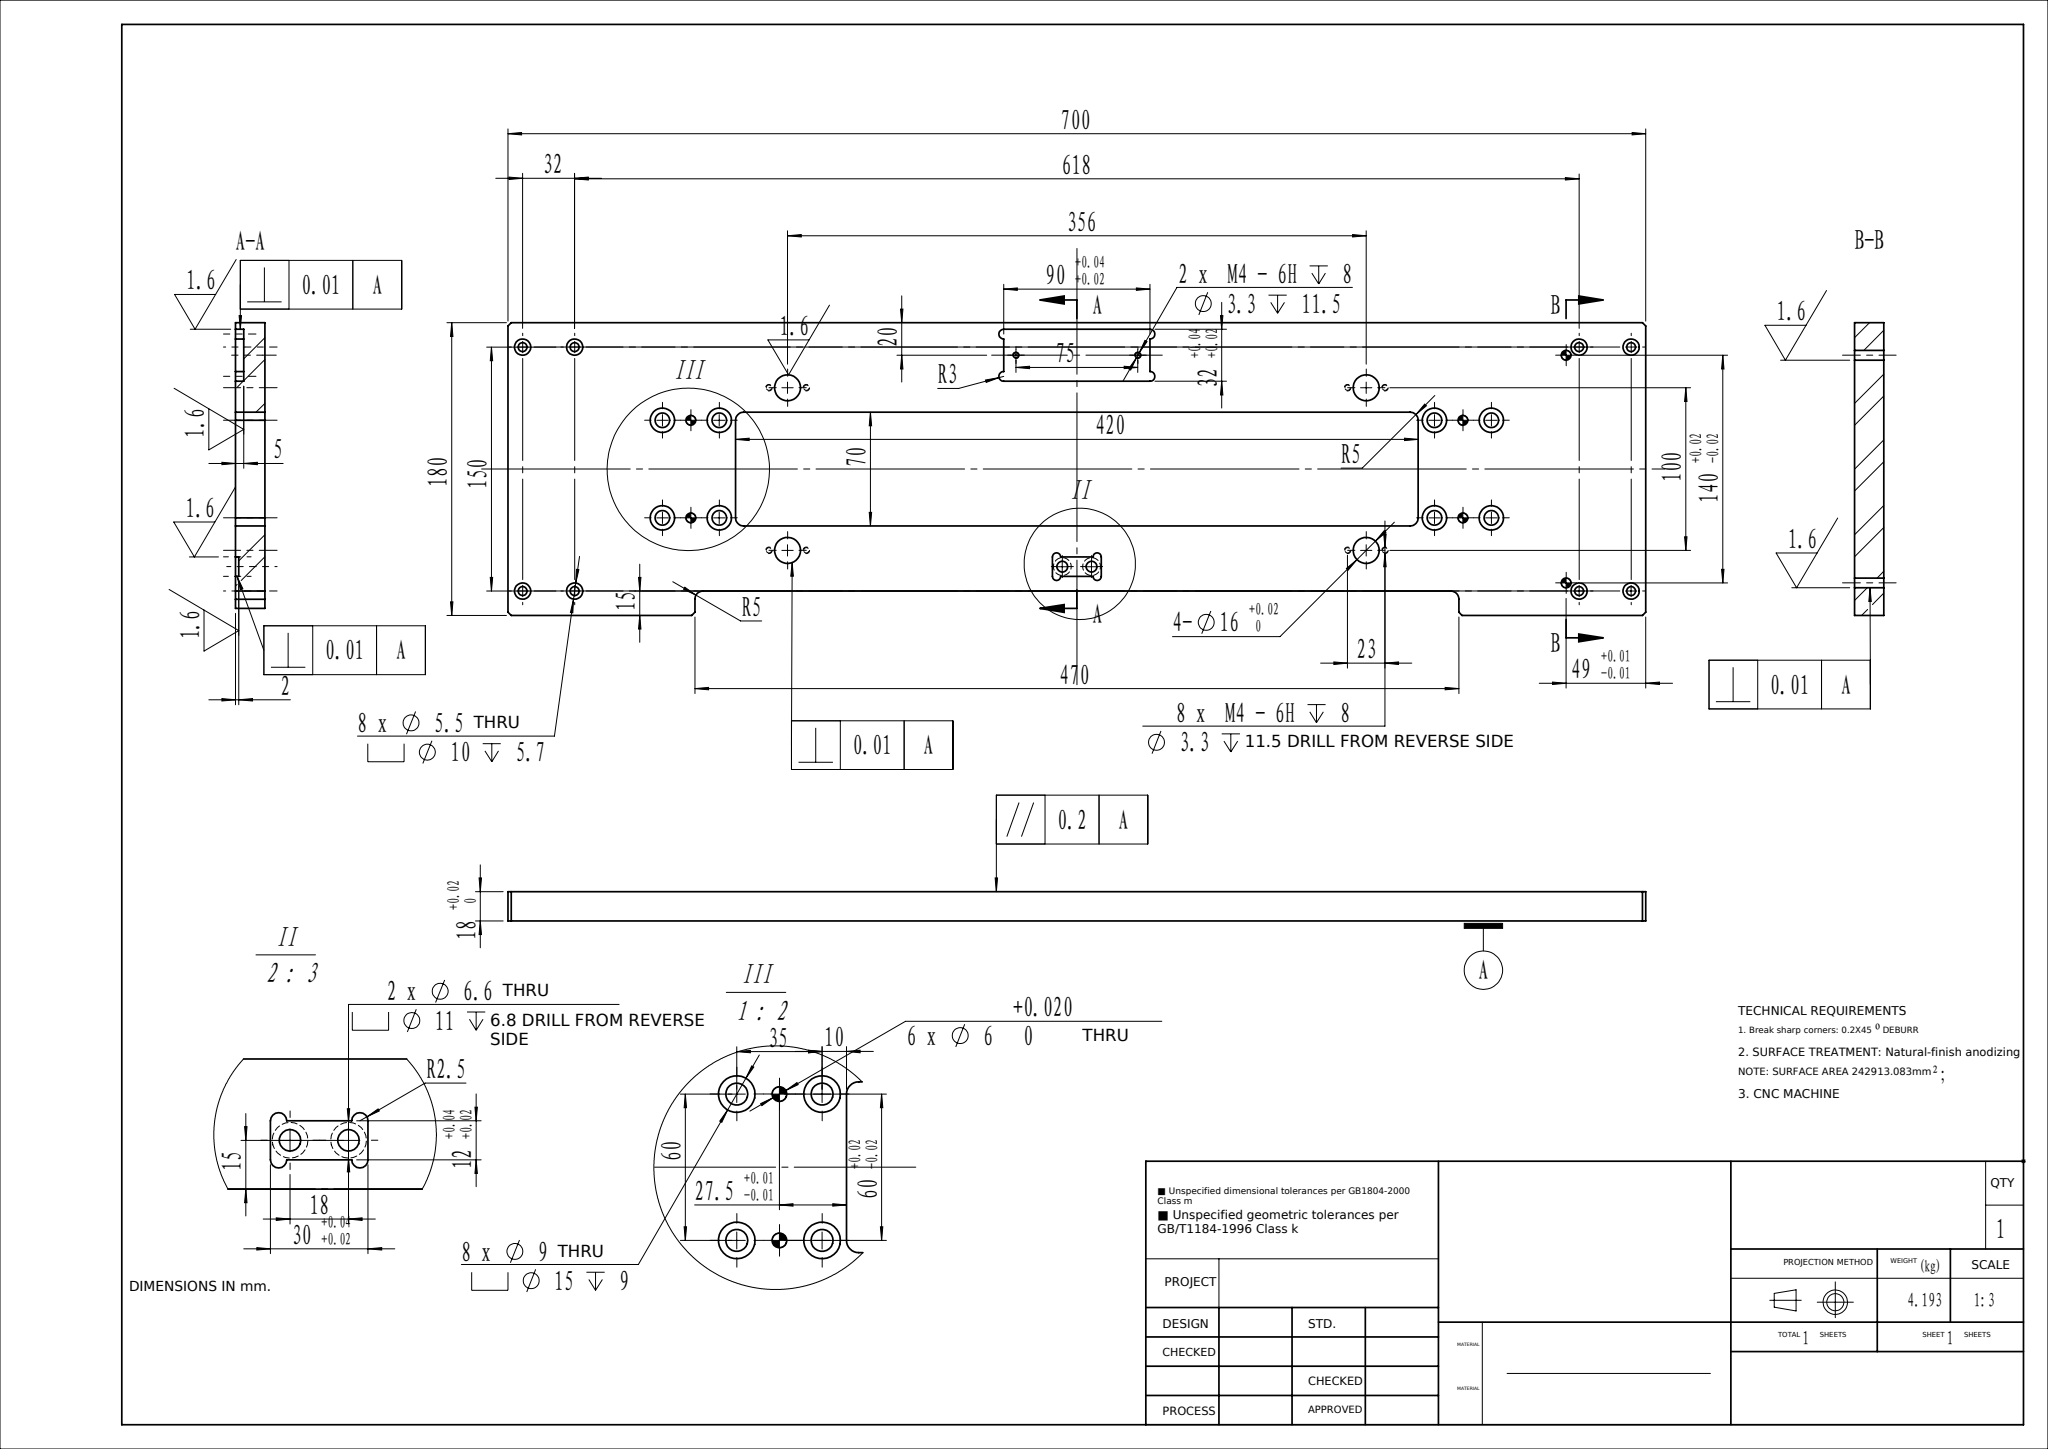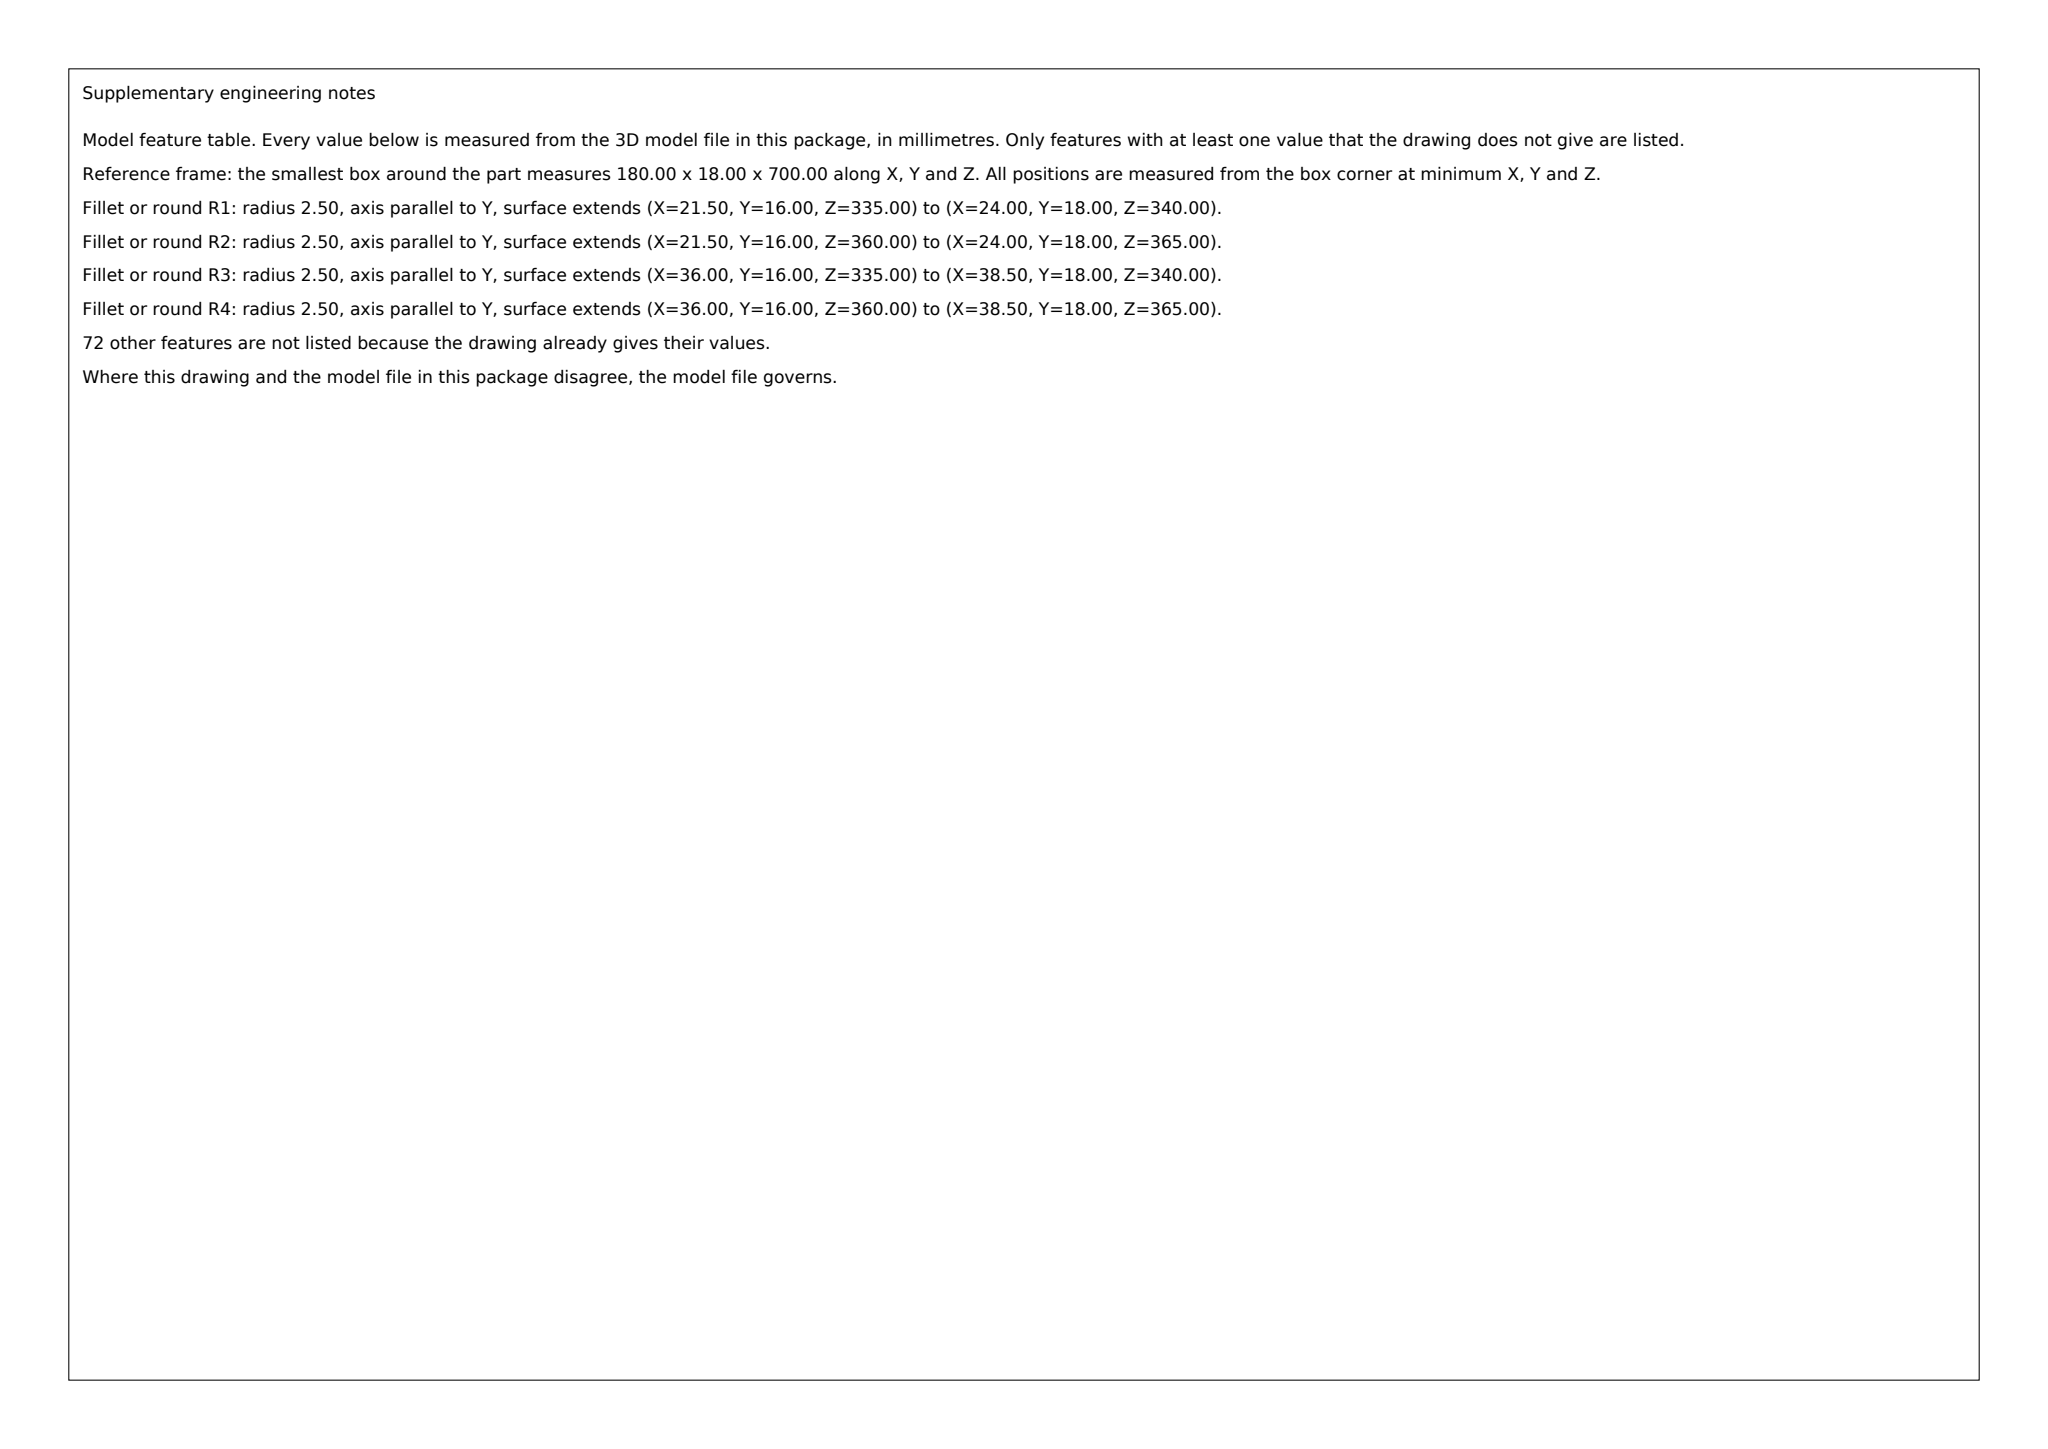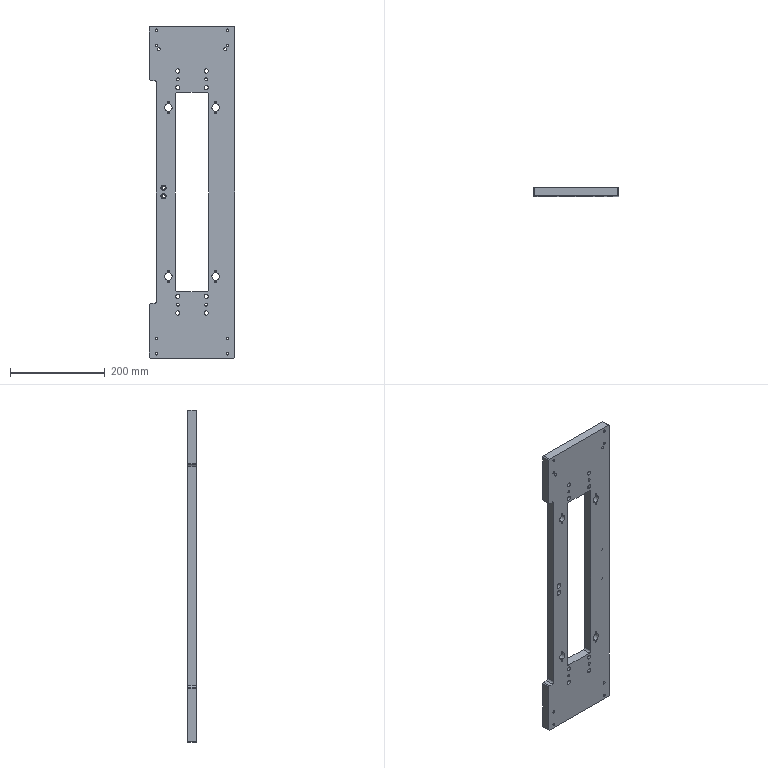Part | SolidWorks | mm | 1 solid | 196 faces | box 180 x 18 x 700 mm | volume 1553095 mm3 | cylinder 128 | plane 48 | cone 20 | commonest cylinder face diameters 10 x22 3.3 x20 6 x18 5.5 x16 15 x16 9 x16 16 x8 11 x4
build123d program:
from build123d import *

# Parameters (mm, degrees)
SKETCH1_W                                            = 180
SKETCH1_H                                            = 700
BOSS_EXTRUDE1_DEPTH                                  = 18
HOLE_SIZE_ACCORDING_TO_THE_TYPE_OF_HEXAG_D           = 9
HOLE_SIZE_ACCORDING_TO_THE_TYPE_OF_HEXAG_CBORE_D     = 15
HOLE_SIZE_ACCORDING_TO_THE_TYPE_OF_HEXAG_CBORE_DEPTH = 9
SKETCH7_W                                            = 70
SKETCH7_H                                            = 420
CUT_EXTRUDE1_DEPTH                                   = 362.834
FILLET1_R                                            = 5
F_16_0_16_DIAMETER_HOLE1_D                           = 16
CIRPATTERN1_COUNT                                    = 2
SKETCH17_W                                           = 15
SKETCH17_H                                           = 470
CUT_EXTRUDE2_DEPTH                                   = 362.834
SKETCH18_R                                           = 3
SKETCH18_W                                           = 32
SKETCH18_H                                           = 90
CUT_EXTRUDE3_DEPTH                                   = 5
M4_TAPPED_HOLE2_D                                    = 3.3
M4_TAPPED_HOLE2_DEPTH                                = 11.5
M4_TAPPED_HOLE2_TIP                                  = 0.9914
CHAMFER1_SIZE                                        = 2
CHAMFER2_SIZE                                        = 2
FILLET2_R                                            = 5
HOLE_SIZE_ACCORDING_TO_THE_TYPE_OF_H_2_D             = 5.5
HOLE_SIZE_ACCORDING_TO_THE_TYPE_OF_H_2_CBORE_D       = 10
HOLE_SIZE_ACCORDING_TO_THE_TYPE_OF_H_2_CBORE_DEPTH   = 5.7
LPATTERN1_COUNT                                      = 2
LPATTERN1_PITCH                                      = 150
LPATTERN1_COUNT_DIR2                                 = 2
LPATTERN1_PITCH_DIR2                                 = 650
F_6_0_6_DIAMETER_HOLE2_D                             = 6
F_6_0_6_DIAMETER_HOLE3_D                             = 6
SKETCH34_R                                           = 2.5
SKETCH34_W                                           = 12
SKETCH34_H                                           = 30
CUT_EXTRUDE4_DEPTH                                   = 2
HOLE_SIZE_ACCORDING_TO_THE_TYPE_OF_H_3_D             = 6.6
HOLE_SIZE_ACCORDING_TO_THE_TYPE_OF_H_3_CBORE_D       = 11
HOLE_SIZE_ACCORDING_TO_THE_TYPE_OF_H_3_CBORE_DEPTH   = 6.8


with BuildPart() as part:
    # Sketch1 → Boss-Extrude1 (new body)
    with BuildSketch(Plane(origin=(0, 0, 0), x_dir=(1, 0, 0), z_dir=(0, 1, 0))):
        Rectangle(SKETCH1_W, SKETCH1_H)
    extrude(amount=BOSS_EXTRUDE1_DEPTH)

    # Hole Size according to the type of Hexag (through all)
    with Locations(Plane(origin=(0, 18, 0), x_dir=(1, 0, 0), z_dir=(0, 1, 0))):
        with Locations((-30, 255), (-30, 220), (30, 255), (30, 220), (-30, -220), (-30, -255), (30, -220), (30, -255)):
            CounterBoreHole(HOLE_SIZE_ACCORDING_TO_THE_TYPE_OF_HEXAG_D / 2, HOLE_SIZE_ACCORDING_TO_THE_TYPE_OF_HEXAG_CBORE_D / 2, HOLE_SIZE_ACCORDING_TO_THE_TYPE_OF_HEXAG_CBORE_DEPTH)

    # Sketch7 → Cut-Extrude1 (cut, through all)
    with BuildSketch(Plane(origin=(0, 18, 0), x_dir=(1, 0, 0), z_dir=(0, 1, 0))):
        Rectangle(SKETCH7_W, SKETCH7_H)
    extrude(amount=-CUT_EXTRUDE1_DEPTH, mode=Mode.SUBTRACT)

    # Fillet1
    fillet1_edges = [part.edges().sort_by_distance(p)[0] for p in [
        (35, 9, -210),
        (35, 9, 210),
        (-35, 9, 210),
        (-35, 9, -210),
    ]]
    fillet(fillet1_edges, radius=FILLET1_R)

    # 16.0 _16_ Diameter Hole1 (through all)
    with Locations(Plane(origin=(0, 18, 0), x_dir=(1, 0, 0), z_dir=(0, 1, 0))):
        with Locations((-50, 178), (50, 178), (-50, -178), (50, -178)):
            Hole(F_16_0_16_DIAMETER_HOLE1_D / 2)

    # Sketch13 → M4 Tapped Hole1 (revolve, cut)
    with BuildSketch(Plane(origin=(50, 0, -189.5), x_dir=(0, 0, -1), z_dir=(1, 0, 0))):
        Polygon((0, 0), (0, 12.491), (1.65, 11.5), (1.65, 0), align=None)
    m4_tapped_hole1 = revolve(axis=Axis((50, -6.35, -189.5), (0, 1, 0)), mode=Mode.SUBTRACT)

    # CirPattern1: M4 Tapped Hole1 ×2 about axis
    cirpattern1_axis = Axis((50, 0, -178), (0, 1, 0))
    for i in range(1, CIRPATTERN1_COUNT):
        add(m4_tapped_hole1.rotate(cirpattern1_axis, i * 360 / CIRPATTERN1_COUNT), mode=Mode.SUBTRACT)

    # Mirror1: M4 Tapped Hole1 across plane
    add(m4_tapped_hole1.mirror(Plane(origin=(0, 0, 0), x_dir=(0, 0, 1), z_dir=(1, 0, 0))), mode=Mode.SUBTRACT)

    # Mirror1 copy 1 sketch → Mirror1 copy 1 (revolve, cut)
    with BuildSketch(Plane(origin=(-50, 0, -166.5), x_dir=(0, 0, 1), z_dir=(1, 0, 0))):
        Polygon((0, 0), (0, -12.491), (1.65, -11.5), (1.65, 0), align=None)
    revolve(axis=Axis((-50, -6.35, -166.5), (0, -1, 0)), mode=Mode.SUBTRACT)

    # Mirror2: M4 Tapped Hole1 across plane
    add(m4_tapped_hole1.mirror(Plane.XY), mode=Mode.SUBTRACT)

    # Mirror2 copy 1 sketch → Mirror2 copy 1 (revolve, cut)
    with BuildSketch(Plane(origin=(50, 0, 166.5), x_dir=(0, 0, -1), z_dir=(-1, 0, 0))):
        Polygon((0, 0), (0, -12.491), (1.65, -11.5), (1.65, 0), align=None)
    revolve(axis=Axis((50, -6.35, 166.5), (0, -1, 0)), mode=Mode.SUBTRACT)

    # Mirror2 copy 2 sketch → Mirror2 copy 2 (revolve, cut)
    with BuildSketch(Plane(origin=(-50, 0, 189.5), x_dir=(0, 0, 1), z_dir=(-1, 0, 0))):
        Polygon((0, 0), (0, 12.491), (1.65, 11.5), (1.65, 0), align=None)
    revolve(axis=Axis((-50, -6.35, 189.5), (0, 1, 0)), mode=Mode.SUBTRACT)

    # Mirror2 copy 3 sketch → Mirror2 copy 3 (revolve, cut)
    with BuildSketch(Plane(origin=(-50, 0, 166.5), x_dir=(0, 0, -1), z_dir=(1, 0, 0))):
        Polygon((0, 0), (0, 12.491), (1.65, 11.5), (1.65, 0), align=None)
    revolve(axis=Axis((-50, -6.35, 166.5), (0, 1, 0)), mode=Mode.SUBTRACT)

    # Sketch17 → Cut-Extrude2 (cut, through all)
    with BuildSketch(Plane(origin=(0, 18, 0), x_dir=(1, 0, 0), z_dir=(0, 1, 0))):
        with Locations((-82.5, 0)):
            Rectangle(SKETCH17_W, SKETCH17_H)
    extrude(amount=-CUT_EXTRUDE2_DEPTH, mode=Mode.SUBTRACT)

    # Sketch18 → Cut-Extrude3 (cut)
    with BuildSketch(Plane(origin=(0, 18, 0), x_dir=(1, 0, 0), z_dir=(0, 1, 0))):
        with Locations((57, 45)):
            Circle(SKETCH18_R)
        with Locations((83, 45)):
            Circle(SKETCH18_R)
        with Locations((57, -45)):
            Circle(SKETCH18_R)
        with Locations((83, -45)):
            Circle(SKETCH18_R)
        with Locations((70, 0)):
            Rectangle(SKETCH18_W, SKETCH18_H)
    extrude(amount=-CUT_EXTRUDE3_DEPTH, mode=Mode.SUBTRACT)

    # M4 Tapped Hole2
    with Locations(Plane(origin=(0, 13, 0), x_dir=(1, 0, 0), z_dir=(0, 1, 0))):
        with Locations((70, 37.5), (70, -37.5)):
            Hole(M4_TAPPED_HOLE2_D / 2, depth=M4_TAPPED_HOLE2_DEPTH)
            with Locations((0, 0, -(M4_TAPPED_HOLE2_DEPTH + M4_TAPPED_HOLE2_TIP / 2))):  # 118° drill point
                Cone(0, M4_TAPPED_HOLE2_D / 2, M4_TAPPED_HOLE2_TIP, mode=Mode.SUBTRACT)

    # Chamfer1
    chamfer1_edges = [part.edges().sort_by_distance(p)[0] for p in [
        (90, 9, 350),
        (-90, 9, 350),
        (-90, 9, -350),
        (90, 9, -350),
    ]]
    chamfer(chamfer1_edges, length=CHAMFER1_SIZE)

    # Chamfer2
    chamfer2_edges = [part.edges().sort_by_distance(p)[0] for p in [
        (-90, 9, 235),
        (-90, 9, -235),
    ]]
    chamfer(chamfer2_edges, length=CHAMFER2_SIZE)

    # Fillet2
    fillet2_edges = [part.edges().sort_by_distance(p)[0] for p in [
        (-75, 9, -235),
        (-75, 9, 235),
    ]]
    fillet(fillet2_edges, radius=FILLET2_R)

    # Hole Size according to the type of H 2 (through all)
    with Locations(Plane(origin=(0, 18, 0), x_dir=(1, 0, 0), z_dir=(0, 1, 0))):
        with Locations((75, -309), (75, -341)):
            hole_size_according_to_the_type_of_h_2 = CounterBoreHole(HOLE_SIZE_ACCORDING_TO_THE_TYPE_OF_H_2_D / 2, HOLE_SIZE_ACCORDING_TO_THE_TYPE_OF_H_2_CBORE_D / 2, HOLE_SIZE_ACCORDING_TO_THE_TYPE_OF_H_2_CBORE_DEPTH)

    # LPattern1: Hole Size according to the type of H 2 2 × 2
    with Locations(*[(-i * LPATTERN1_PITCH, 0, -j * LPATTERN1_PITCH_DIR2) for i in range(LPATTERN1_COUNT) for j in range(LPATTERN1_COUNT_DIR2) if (i, j) != (0, 0)]):
        add(hole_size_according_to_the_type_of_h_2, mode=Mode.SUBTRACT)

    # 6.0 _6_ Diameter Hole2 (through all)
    with Locations(Plane(origin=(0, 18, 0), x_dir=(1, 0, 0), z_dir=(0, 1, 0))):
        with Locations((-70, -301), (70, -301)):
            Hole(F_6_0_6_DIAMETER_HOLE2_D / 2)

    # 6.0 _6_ Diameter Hole3 (through all)
    with Locations(Plane(origin=(0, 18, 0), x_dir=(1, 0, 0), z_dir=(0, 1, 0))):
        with Locations((-30, 237.5), (30, 237.5), (-30, -237.5), (30, -237.5)):
            Hole(F_6_0_6_DIAMETER_HOLE3_D / 2)

    # Sketch34 → Cut-Extrude4 (cut)
    with BuildSketch(Plane(origin=(0, 18, 0), x_dir=(1, 0, 0), z_dir=(0, 1, 0))):
        with Locations((-66, 12.5)):
            Circle(SKETCH34_R)
        with Locations((-66, -12.5)):
            Circle(SKETCH34_R)
        with Locations((-54, -12.5)):
            Circle(SKETCH34_R)
        with Locations((-54, 12.5)):
            Circle(SKETCH34_R)
        with Locations((-60, 0)):
            Rectangle(SKETCH34_W, SKETCH34_H)
        with BuildLine():
            ThreePointArc((-66, 15), (-68.5, 12.5), (-66, 10))
            Line((-66, 10), (-66, 15))
        make_face()
        with BuildLine():
            Line((-66, 15), (-66, 10))
            ThreePointArc((-66, 10), (-64.232, 10.732), (-63.5, 12.5))
            ThreePointArc((-63.5, 12.5), (-64.232, 14.268), (-66, 15))
        make_face()
        with BuildLine():
            ThreePointArc((-66, 15), (-68.5, 12.5), (-66, 10))
            Line((-66, 10), (-66, 15))
        make_face()
        with BuildLine():
            Line((-66, 15), (-66, 10))
            ThreePointArc((-66, 10), (-64.232, 10.732), (-63.5, 12.5))
            ThreePointArc((-63.5, 12.5), (-64.232, 14.268), (-66, 15))
        make_face()
        with BuildLine():
            ThreePointArc((-66, -10), (-68.5, -12.5), (-66, -15))
            Line((-66, -15), (-66, -10))
        make_face()
        with BuildLine():
            Line((-66, -10), (-66, -15))
            ThreePointArc((-66, -15), (-64.232, -14.268), (-63.5, -12.5))
            ThreePointArc((-63.5, -12.5), (-64.232, -10.732), (-66, -10))
        make_face()
        with BuildLine():
            ThreePointArc((-66, -10), (-68.5, -12.5), (-66, -15))
            Line((-66, -15), (-66, -10))
        make_face()
        with BuildLine():
            Line((-66, -10), (-66, -15))
            ThreePointArc((-66, -15), (-64.232, -14.268), (-63.5, -12.5))
            ThreePointArc((-63.5, -12.5), (-64.232, -10.732), (-66, -10))
        make_face()
        with BuildLine():
            ThreePointArc((-54, -10), (-56.5, -12.5), (-54, -15))
            Line((-54, -15), (-54, -10))
        make_face()
        with BuildLine():
            Line((-54, -10), (-54, -15))
            ThreePointArc((-54, -15), (-52.232, -14.268), (-51.5, -12.5))
            ThreePointArc((-51.5, -12.5), (-52.232, -10.732), (-54, -10))
        make_face()
        with BuildLine():
            ThreePointArc((-54, -10), (-56.5, -12.5), (-54, -15))
            Line((-54, -15), (-54, -10))
        make_face()
        with BuildLine():
            Line((-54, -10), (-54, -15))
            ThreePointArc((-54, -15), (-52.232, -14.268), (-51.5, -12.5))
            ThreePointArc((-51.5, -12.5), (-52.232, -10.732), (-54, -10))
        make_face()
        with BuildLine():
            ThreePointArc((-54, 15), (-56.5, 12.5), (-54, 10))
            Line((-54, 10), (-54, 15))
        make_face()
        with BuildLine():
            Line((-54, 15), (-54, 10))
            ThreePointArc((-54, 10), (-52.232, 10.732), (-51.5, 12.5))
            ThreePointArc((-51.5, 12.5), (-52.232, 14.268), (-54, 15))
        make_face()
        with BuildLine():
            ThreePointArc((-54, 15), (-56.5, 12.5), (-54, 10))
            Line((-54, 10), (-54, 15))
        make_face()
        with BuildLine():
            Line((-54, 15), (-54, 10))
            ThreePointArc((-54, 10), (-52.232, 10.732), (-51.5, 12.5))
            ThreePointArc((-51.5, 12.5), (-52.232, 14.268), (-54, 15))
        make_face()
    extrude(amount=-CUT_EXTRUDE4_DEPTH, mode=Mode.SUBTRACT)

    # Hole Size according to the type of H 3 (through all)
    with Locations(Plane(origin=(0, 0, 0), x_dir=(-1, 0, 0), z_dir=(0, -1, 0))):
        with Locations((60, -9), (60, 9)):
            CounterBoreHole(HOLE_SIZE_ACCORDING_TO_THE_TYPE_OF_H_3_D / 2, HOLE_SIZE_ACCORDING_TO_THE_TYPE_OF_H_3_CBORE_D / 2, HOLE_SIZE_ACCORDING_TO_THE_TYPE_OF_H_3_CBORE_DEPTH)


solid = part.part